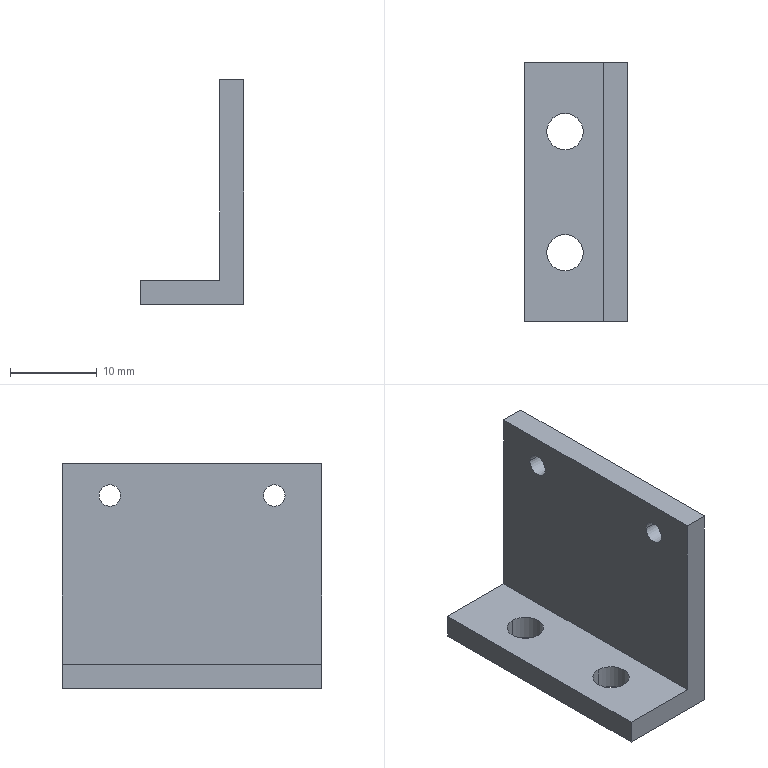Component | SolidWorks | 6G-DCSG-ZeroPointSwitchSeat-1 | 1 solid | 16 faces | box 12 x 30 x 26 mm | volume 2852 mm3 | cylinder 8 | plane 8 | commonest cylinder face diameters 2.5 x4 4.2 x4
build123d program:
from build123d import *

# Parameters (mm, degrees)
BOSS_EXTRUDE1_DEPTH = 15
SKETCH2_R           = 2.1
CUT_EXTRUDE1_DEPTH  = 30
M3_TAPPED_HOLE1_D   = 2.5
SKETCH5_W           = 7.11
SKETCH5_H           = 30
CUT_EXTRUDE2_DEPTH  = 24.497


with BuildPart() as part:
    # Sketch1 → Boss-Extrude1 (new, symmetric)
    with BuildSketch(Plane.XY):
        Polygon((-14.429, 2.972), (12.771, 2.972), (12.771, -6.228), (15.571, -6.228), (15.571, 5.772), (-14.429, 5.772), align=None)
    extrude(amount=BOSS_EXTRUDE1_DEPTH, both=True)

    # Sketch2 → Cut-Extrude1 (cut)
    with BuildSketch(Plane.ZY.offset(-12.771)):
        with Locations((-7, -1.5)):
            Circle(SKETCH2_R)
        with Locations((7, -1.5)):
            Circle(SKETCH2_R)
    extrude(amount=-CUT_EXTRUDE1_DEPTH, mode=Mode.SUBTRACT)

    # M3 Tapped Hole1 (through all)
    with Locations(Plane(origin=(-6.729, 2.972, 9.5), x_dir=(-1, 0, 0), z_dir=(0, -1, 0))):
        with Locations((0, 0), (0, 18.993)):
            Hole(M3_TAPPED_HOLE1_D / 2)

    # Sketch5 → Cut-Extrude2 (cut, through all)
    with BuildSketch(Plane.XZ.offset(-2.972)):
        with Locations((-13.984, 0)):
            Rectangle(SKETCH5_W, SKETCH5_H)
    extrude(amount=-CUT_EXTRUDE2_DEPTH, mode=Mode.SUBTRACT)


solid = part.part

# Placed as in the assembly
solid = solid.moved(Location((181.5, -79, 15.571), (90, 0, -90)))
STEP:
#1=COLOUR_RGB('',0.7922,0.8196,0.9333);
#2=FILL_AREA_STYLE_COLOUR('',#1);
#3=FILL_AREA_STYLE('',(#2));
#4=SURFACE_STYLE_FILL_AREA(#3);
#5=SURFACE_SIDE_STYLE('',(#4));
#6=SURFACE_STYLE_USAGE(.BOTH.,#5);
#7=PRESENTATION_STYLE_ASSIGNMENT((#6));
#8=CARTESIAN_POINT('',(7.373,-3.533,0.878));
#9=VERTEX_POINT('',#8);
#10=CARTESIAN_POINT('',(7.373,-3.435,0.878));
#11=VERTEX_POINT('',#10);
#12=CARTESIAN_POINT('',(7.373,-3.484,0.878));
#13=DIRECTION('',(-1.,-0.,0.));
#14=DIRECTION('',(0.,1.,0.));
#15=AXIS2_PLACEMENT_3D('',#12,#13,#14);
#16=CIRCLE('',#15,0.04921);
#17=EDGE_CURVE('',#9,#11,#16,.T.);
#18=ORIENTED_EDGE('',*,*,#17,.F.);
#19=CARTESIAN_POINT('',(7.263,-3.533,0.878));
#20=VERTEX_POINT('',#19);
#21=CARTESIAN_POINT('',(7.263,-3.533,0.878));
#22=DIRECTION('',(-1.,-0.,0.));
#23=VECTOR('',#22,39.37);
#24=LINE('',#21,#23);
#25=EDGE_CURVE('',#9,#20,#24,.T.);
#26=ORIENTED_EDGE('',*,*,#25,.T.);
#27=CARTESIAN_POINT('',(7.263,-3.435,0.878));
#28=VERTEX_POINT('',#27);
#29=CARTESIAN_POINT('',(7.263,-3.484,0.878));
#30=DIRECTION('',(-1.,-0.,0.));
#31=DIRECTION('',(0.,1.,0.));
#32=AXIS2_PLACEMENT_3D('',#29,#30,#31);
#33=CIRCLE('',#32,0.04921);
#34=EDGE_CURVE('',#20,#28,#33,.T.);
#35=ORIENTED_EDGE('',*,*,#34,.T.);
#36=CARTESIAN_POINT('',(7.263,-3.435,0.878));
#37=DIRECTION('',(-1.,-0.,0.));
#38=VECTOR('',#37,39.37);
#39=LINE('',#36,#38);
#40=EDGE_CURVE('',#11,#28,#39,.T.);
#41=ORIENTED_EDGE('',*,*,#40,.F.);
#42=EDGE_LOOP('',(#18,#26,#35,#41));
#43=FACE_OUTER_BOUND('',#42,.T.);
#44=CARTESIAN_POINT('',(7.263,-3.484,0.878));
#45=DIRECTION('',(-1.,-0.,0.));
#46=DIRECTION('',(0.,1.,0.));
#47=AXIS2_PLACEMENT_3D('',#44,#45,#46);
#48=CYLINDRICAL_SURFACE('',#47,0.04921);
#49=ADVANCED_FACE('',(#43),#48,.F.);
#50=CARTESIAN_POINT('',(7.373,-2.786,0.878));
#51=VERTEX_POINT('',#50);
#52=CARTESIAN_POINT('',(7.373,-2.687,0.878));
#53=VERTEX_POINT('',#52);
#54=CARTESIAN_POINT('',(7.373,-2.737,0.878));
#55=DIRECTION('',(-1.,-0.,0.));
#56=DIRECTION('',(0.,1.,0.));
#57=AXIS2_PLACEMENT_3D('',#54,#55,#56);
#58=CIRCLE('',#57,0.04921);
#59=EDGE_CURVE('',#51,#53,#58,.T.);
#60=ORIENTED_EDGE('',*,*,#59,.F.);
#61=CARTESIAN_POINT('',(7.263,-2.786,0.878));
#62=VERTEX_POINT('',#61);
#63=CARTESIAN_POINT('',(7.263,-2.786,0.878));
#64=DIRECTION('',(-1.,-0.,0.));
#65=VECTOR('',#64,39.37);
#66=LINE('',#63,#65);
#67=EDGE_CURVE('',#51,#62,#66,.T.);
#68=ORIENTED_EDGE('',*,*,#67,.T.);
#69=CARTESIAN_POINT('',(7.263,-2.687,0.878));
#70=VERTEX_POINT('',#69);
#71=CARTESIAN_POINT('',(7.263,-2.737,0.878));
#72=DIRECTION('',(-1.,-0.,0.));
#73=DIRECTION('',(0.,1.,0.));
#74=AXIS2_PLACEMENT_3D('',#71,#72,#73);
#75=CIRCLE('',#74,0.04921);
#76=EDGE_CURVE('',#62,#70,#75,.T.);
#77=ORIENTED_EDGE('',*,*,#76,.T.);
#78=CARTESIAN_POINT('',(7.263,-2.687,0.878));
#79=DIRECTION('',(-1.,-0.,0.));
#80=VECTOR('',#79,39.37);
#81=LINE('',#78,#80);
#82=EDGE_CURVE('',#53,#70,#81,.T.);
#83=ORIENTED_EDGE('',*,*,#82,.F.);
#84=EDGE_LOOP('',(#60,#68,#77,#83));
#85=FACE_OUTER_BOUND('',#84,.T.);
#86=CARTESIAN_POINT('',(7.263,-2.737,0.878));
#87=DIRECTION('',(-1.,-0.,0.));
#88=DIRECTION('',(0.,1.,0.));
#89=AXIS2_PLACEMENT_3D('',#86,#87,#88);
#90=CYLINDRICAL_SURFACE('',#89,0.04921);
#91=ADVANCED_FACE('',(#85),#90,.F.);
#92=CARTESIAN_POINT('',(7.087,-3.303,0.));
#93=VERTEX_POINT('',#92);
#94=CARTESIAN_POINT('',(7.087,-3.469,0.));
#95=VERTEX_POINT('',#94);
#96=CARTESIAN_POINT('',(7.087,-3.386,0.));
#97=DIRECTION('',(0.,0.,1.));
#98=DIRECTION('',(0.,-1.,0.));
#99=AXIS2_PLACEMENT_3D('',#96,#97,#98);
#100=CIRCLE('',#99,0.08268);
#101=EDGE_CURVE('',#93,#95,#100,.T.);
#102=ORIENTED_EDGE('',*,*,#101,.F.);
#103=CARTESIAN_POINT('',(7.087,-3.303,0.1102));
#104=VERTEX_POINT('',#103);
#105=CARTESIAN_POINT('',(7.087,-3.303,-1.071));
#106=DIRECTION('',(0.,0.,1.));
#107=VECTOR('',#106,39.37);
#108=LINE('',#105,#107);
#109=EDGE_CURVE('',#93,#104,#108,.T.);
#110=ORIENTED_EDGE('',*,*,#109,.T.);
#111=CARTESIAN_POINT('',(7.087,-3.469,0.1102));
#112=VERTEX_POINT('',#111);
#113=CARTESIAN_POINT('',(7.087,-3.386,0.1102));
#114=DIRECTION('',(0.,0.,1.));
#115=DIRECTION('',(0.,-1.,0.));
#116=AXIS2_PLACEMENT_3D('',#113,#114,#115);
#117=CIRCLE('',#116,0.08268);
#118=EDGE_CURVE('',#104,#112,#117,.T.);
#119=ORIENTED_EDGE('',*,*,#118,.T.);
#120=CARTESIAN_POINT('',(7.087,-3.469,-1.071));
#121=DIRECTION('',(0.,0.,1.));
#122=VECTOR('',#121,39.37);
#123=LINE('',#120,#122);
#124=EDGE_CURVE('',#95,#112,#123,.T.);
#125=ORIENTED_EDGE('',*,*,#124,.F.);
#126=EDGE_LOOP('',(#102,#110,#119,#125));
#127=FACE_OUTER_BOUND('',#126,.T.);
#128=CARTESIAN_POINT('',(7.087,-3.386,-1.071));
#129=DIRECTION('',(0.,0.,1.));
#130=DIRECTION('',(0.,-1.,0.));
#131=AXIS2_PLACEMENT_3D('',#128,#129,#130);
#132=CYLINDRICAL_SURFACE('',#131,0.08268);
#133=ADVANCED_FACE('',(#127),#132,.F.);
#134=CARTESIAN_POINT('',(7.087,-2.752,0.));
#135=VERTEX_POINT('',#134);
#136=CARTESIAN_POINT('',(7.087,-2.917,0.));
#137=VERTEX_POINT('',#136);
#138=CARTESIAN_POINT('',(7.087,-2.835,0.));
#139=DIRECTION('',(0.,0.,1.));
#140=DIRECTION('',(0.,-1.,0.));
#141=AXIS2_PLACEMENT_3D('',#138,#139,#140);
#142=CIRCLE('',#141,0.08268);
#143=EDGE_CURVE('',#135,#137,#142,.T.);
#144=ORIENTED_EDGE('',*,*,#143,.F.);
#145=CARTESIAN_POINT('',(7.087,-2.752,0.1102));
#146=VERTEX_POINT('',#145);
#147=CARTESIAN_POINT('',(7.087,-2.752,-1.071));
#148=DIRECTION('',(0.,0.,1.));
#149=VECTOR('',#148,39.37);
#150=LINE('',#147,#149);
#151=EDGE_CURVE('',#135,#146,#150,.T.);
#152=ORIENTED_EDGE('',*,*,#151,.T.);
#153=CARTESIAN_POINT('',(7.087,-2.917,0.1102));
#154=VERTEX_POINT('',#153);
#155=CARTESIAN_POINT('',(7.087,-2.835,0.1102));
#156=DIRECTION('',(0.,0.,1.));
#157=DIRECTION('',(0.,-1.,0.));
#158=AXIS2_PLACEMENT_3D('',#155,#156,#157);
#159=CIRCLE('',#158,0.08268);
#160=EDGE_CURVE('',#146,#154,#159,.T.);
#161=ORIENTED_EDGE('',*,*,#160,.T.);
#162=CARTESIAN_POINT('',(7.087,-2.917,-1.071));
#163=DIRECTION('',(0.,0.,1.));
#164=VECTOR('',#163,39.37);
#165=LINE('',#162,#164);
#166=EDGE_CURVE('',#137,#154,#165,.T.);
#167=ORIENTED_EDGE('',*,*,#166,.F.);
#168=EDGE_LOOP('',(#144,#152,#161,#167));
#169=FACE_OUTER_BOUND('',#168,.T.);
#170=CARTESIAN_POINT('',(7.087,-2.835,-1.071));
#171=DIRECTION('',(0.,0.,1.));
#172=DIRECTION('',(0.,-1.,0.));
#173=AXIS2_PLACEMENT_3D('',#170,#171,#172);
#174=CYLINDRICAL_SURFACE('',#173,0.08268);
#175=ADVANCED_FACE('',(#169),#174,.F.);
#176=CARTESIAN_POINT('',(7.087,-3.386,0.));
#177=DIRECTION('',(0.,0.,1.));
#178=DIRECTION('',(0.,-1.,0.));
#179=AXIS2_PLACEMENT_3D('',#176,#177,#178);
#180=CIRCLE('',#179,0.08268);
#181=EDGE_CURVE('',#95,#93,#180,.T.);
#182=ORIENTED_EDGE('',*,*,#181,.T.);
#183=ORIENTED_EDGE('',*,*,#101,.T.);
#184=EDGE_LOOP('',(#182,#183));
#185=FACE_BOUND('',#184,.T.);
#186=CARTESIAN_POINT('',(7.087,-2.835,0.));
#187=DIRECTION('',(0.,0.,1.));
#188=DIRECTION('',(0.,-1.,0.));
#189=AXIS2_PLACEMENT_3D('',#186,#187,#188);
#190=CIRCLE('',#189,0.08268);
#191=EDGE_CURVE('',#137,#135,#190,.T.);
#192=ORIENTED_EDGE('',*,*,#191,.T.);
#193=ORIENTED_EDGE('',*,*,#143,.T.);
#194=EDGE_LOOP('',(#192,#193));
#195=FACE_BOUND('',#194,.T.);
#196=CARTESIAN_POINT('',(6.9,-2.52,0.));
#197=VERTEX_POINT('',#196);
#198=CARTESIAN_POINT('',(7.373,-2.52,0.));
#199=VERTEX_POINT('',#198);
#200=CARTESIAN_POINT('',(6.9,-2.52,0.));
#201=DIRECTION('',(1.,0.,-0.));
#202=VECTOR('',#201,39.37);
#203=LINE('',#200,#202);
#204=EDGE_CURVE('',#197,#199,#203,.T.);
#205=ORIENTED_EDGE('',*,*,#204,.T.);
#206=CARTESIAN_POINT('',(7.373,-3.701,0.));
#207=VERTEX_POINT('',#206);
#208=CARTESIAN_POINT('',(7.373,-3.701,0.));
#209=DIRECTION('',(-0.,1.,0.));
#210=VECTOR('',#209,39.37);
#211=LINE('',#208,#210);
#212=EDGE_CURVE('',#207,#199,#211,.T.);
#213=ORIENTED_EDGE('',*,*,#212,.F.);
#214=CARTESIAN_POINT('',(6.9,-3.701,0.));
#215=VERTEX_POINT('',#214);
#216=CARTESIAN_POINT('',(6.9,-3.701,0.));
#217=DIRECTION('',(1.,0.,-0.));
#218=VECTOR('',#217,39.37);
#219=LINE('',#216,#218);
#220=EDGE_CURVE('',#215,#207,#219,.T.);
#221=ORIENTED_EDGE('',*,*,#220,.F.);
#222=CARTESIAN_POINT('',(6.9,-3.701,0.));
#223=DIRECTION('',(-0.,1.,0.));
#224=VECTOR('',#223,39.37);
#225=LINE('',#222,#224);
#226=EDGE_CURVE('',#215,#197,#225,.T.);
#227=ORIENTED_EDGE('',*,*,#226,.T.);
#228=EDGE_LOOP('',(#205,#213,#221,#227));
#229=FACE_OUTER_BOUND('',#228,.T.);
#230=CARTESIAN_POINT('',(6.9,-3.701,0.));
#231=DIRECTION('',(0.,0.,1.));
#232=DIRECTION('',(0.,-1.,0.));
#233=AXIS2_PLACEMENT_3D('',#230,#231,#232);
#234=PLANE('',#233);
#235=ADVANCED_FACE('',(#185,#195,#229),#234,.F.);
#236=CARTESIAN_POINT('',(7.373,-3.484,0.878));
#237=DIRECTION('',(-1.,-0.,0.));
#238=DIRECTION('',(0.,1.,0.));
#239=AXIS2_PLACEMENT_3D('',#236,#237,#238);
#240=CIRCLE('',#239,0.04921);
#241=EDGE_CURVE('',#11,#9,#240,.T.);
#242=ORIENTED_EDGE('',*,*,#241,.T.);
#243=ORIENTED_EDGE('',*,*,#17,.T.);
#244=EDGE_LOOP('',(#242,#243));
#245=FACE_BOUND('',#244,.T.);
#246=CARTESIAN_POINT('',(7.373,-2.737,0.878));
#247=DIRECTION('',(-1.,-0.,0.));
#248=DIRECTION('',(0.,1.,0.));
#249=AXIS2_PLACEMENT_3D('',#246,#247,#248);
#250=CIRCLE('',#249,0.04921);
#251=EDGE_CURVE('',#53,#51,#250,.T.);
#252=ORIENTED_EDGE('',*,*,#251,.T.);
#253=ORIENTED_EDGE('',*,*,#59,.T.);
#254=EDGE_LOOP('',(#252,#253));
#255=FACE_BOUND('',#254,.T.);
#256=CARTESIAN_POINT('',(7.373,-2.52,1.024));
#257=VERTEX_POINT('',#256);
#258=CARTESIAN_POINT('',(7.373,-2.52,1.181));
#259=DIRECTION('',(0.,0.,1.));
#260=VECTOR('',#259,39.37);
#261=LINE('',#258,#260);
#262=EDGE_CURVE('',#199,#257,#261,.T.);
#263=ORIENTED_EDGE('',*,*,#262,.T.);
#264=CARTESIAN_POINT('',(7.373,-3.701,1.024));
#265=VERTEX_POINT('',#264);
#266=CARTESIAN_POINT('',(7.373,-3.701,1.024));
#267=DIRECTION('',(0.,-1.,0.));
#268=VECTOR('',#267,39.37);
#269=LINE('',#266,#268);
#270=EDGE_CURVE('',#257,#265,#269,.T.);
#271=ORIENTED_EDGE('',*,*,#270,.T.);
#272=CARTESIAN_POINT('',(7.373,-3.701,1.181));
#273=DIRECTION('',(0.,0.,1.));
#274=VECTOR('',#273,39.37);
#275=LINE('',#272,#274);
#276=EDGE_CURVE('',#207,#265,#275,.T.);
#277=ORIENTED_EDGE('',*,*,#276,.F.);
#278=ORIENTED_EDGE('',*,*,#212,.T.);
#279=EDGE_LOOP('',(#263,#271,#277,#278));
#280=FACE_OUTER_BOUND('',#279,.T.);
#281=CARTESIAN_POINT('',(7.373,-3.701,1.181));
#282=DIRECTION('',(-1.,-0.,0.));
#283=DIRECTION('',(-0.,1.,0.));
#284=AXIS2_PLACEMENT_3D('',#281,#282,#283);
#285=PLANE('',#284);
#286=ADVANCED_FACE('',(#245,#255,#280),#285,.F.);
#287=CARTESIAN_POINT('',(7.263,-3.484,0.878));
#288=DIRECTION('',(-1.,-0.,0.));
#289=DIRECTION('',(0.,1.,0.));
#290=AXIS2_PLACEMENT_3D('',#287,#288,#289);
#291=CIRCLE('',#290,0.04921);
#292=EDGE_CURVE('',#28,#20,#291,.T.);
#293=ORIENTED_EDGE('',*,*,#292,.F.);
#294=ORIENTED_EDGE('',*,*,#34,.F.);
#295=EDGE_LOOP('',(#293,#294));
#296=FACE_BOUND('',#295,.T.);
#297=CARTESIAN_POINT('',(7.263,-2.737,0.878));
#298=DIRECTION('',(-1.,-0.,0.));
#299=DIRECTION('',(0.,1.,0.));
#300=AXIS2_PLACEMENT_3D('',#297,#298,#299);
#301=CIRCLE('',#300,0.04921);
#302=EDGE_CURVE('',#70,#62,#301,.T.);
#303=ORIENTED_EDGE('',*,*,#302,.F.);
#304=ORIENTED_EDGE('',*,*,#76,.F.);
#305=EDGE_LOOP('',(#303,#304));
#306=FACE_BOUND('',#305,.T.);
#307=CARTESIAN_POINT('',(7.263,-3.701,1.024));
#308=VERTEX_POINT('',#307);
#309=CARTESIAN_POINT('',(7.263,-3.701,0.1102));
#310=VERTEX_POINT('',#309);
#311=CARTESIAN_POINT('',(7.263,-3.701,1.181));
#312=DIRECTION('',(-0.,-0.,-1.));
#313=VECTOR('',#312,39.37);
#314=LINE('',#311,#313);
#315=EDGE_CURVE('',#308,#310,#314,.T.);
#316=ORIENTED_EDGE('',*,*,#315,.F.);
#317=CARTESIAN_POINT('',(7.263,-2.52,1.024));
#318=VERTEX_POINT('',#317);
#319=CARTESIAN_POINT('',(7.263,-3.701,1.024));
#320=DIRECTION('',(0.,-1.,0.));
#321=VECTOR('',#320,39.37);
#322=LINE('',#319,#321);
#323=EDGE_CURVE('',#318,#308,#322,.T.);
#324=ORIENTED_EDGE('',*,*,#323,.F.);
#325=CARTESIAN_POINT('',(7.263,-2.52,0.1102));
#326=VERTEX_POINT('',#325);
#327=CARTESIAN_POINT('',(7.263,-2.52,1.181));
#328=DIRECTION('',(-0.,-0.,-1.));
#329=VECTOR('',#328,39.37);
#330=LINE('',#327,#329);
#331=EDGE_CURVE('',#318,#326,#330,.T.);
#332=ORIENTED_EDGE('',*,*,#331,.T.);
#333=CARTESIAN_POINT('',(7.263,-3.701,0.1102));
#334=DIRECTION('',(-0.,1.,0.));
#335=VECTOR('',#334,39.37);
#336=LINE('',#333,#335);
#337=EDGE_CURVE('',#310,#326,#336,.T.);
#338=ORIENTED_EDGE('',*,*,#337,.F.);
#339=EDGE_LOOP('',(#316,#324,#332,#338));
#340=FACE_OUTER_BOUND('',#339,.T.);
#341=CARTESIAN_POINT('',(7.263,-3.701,1.181));
#342=DIRECTION('',(1.,0.,-0.));
#343=DIRECTION('',(0.,0.,1.));
#344=AXIS2_PLACEMENT_3D('',#341,#342,#343);
#345=PLANE('',#344);
#346=ADVANCED_FACE('',(#296,#306,#340),#345,.F.);
#347=CARTESIAN_POINT('',(7.087,-3.386,0.1102));
#348=DIRECTION('',(0.,0.,1.));
#349=DIRECTION('',(0.,-1.,0.));
#350=AXIS2_PLACEMENT_3D('',#347,#348,#349);
#351=CIRCLE('',#350,0.08268);
#352=EDGE_CURVE('',#112,#104,#351,.T.);
#353=ORIENTED_EDGE('',*,*,#352,.F.);
#354=ORIENTED_EDGE('',*,*,#118,.F.);
#355=EDGE_LOOP('',(#353,#354));
#356=FACE_BOUND('',#355,.T.);
#357=CARTESIAN_POINT('',(7.087,-2.835,0.1102));
#358=DIRECTION('',(0.,0.,1.));
#359=DIRECTION('',(0.,-1.,0.));
#360=AXIS2_PLACEMENT_3D('',#357,#358,#359);
#361=CIRCLE('',#360,0.08268);
#362=EDGE_CURVE('',#154,#146,#361,.T.);
#363=ORIENTED_EDGE('',*,*,#362,.F.);
#364=ORIENTED_EDGE('',*,*,#160,.F.);
#365=EDGE_LOOP('',(#363,#364));
#366=FACE_BOUND('',#365,.T.);
#367=CARTESIAN_POINT('',(6.9,-2.52,0.1102));
#368=VERTEX_POINT('',#367);
#369=CARTESIAN_POINT('',(6.9,-2.52,0.1102));
#370=DIRECTION('',(-1.,-0.,0.));
#371=VECTOR('',#370,39.37);
#372=LINE('',#369,#371);
#373=EDGE_CURVE('',#326,#368,#372,.T.);
#374=ORIENTED_EDGE('',*,*,#373,.T.);
#375=CARTESIAN_POINT('',(6.9,-3.701,0.1102));
#376=VERTEX_POINT('',#375);
#377=CARTESIAN_POINT('',(6.9,-3.701,0.1102));
#378=DIRECTION('',(-0.,1.,0.));
#379=VECTOR('',#378,39.37);
#380=LINE('',#377,#379);
#381=EDGE_CURVE('',#376,#368,#380,.T.);
#382=ORIENTED_EDGE('',*,*,#381,.F.);
#383=CARTESIAN_POINT('',(6.9,-3.701,0.1102));
#384=DIRECTION('',(-1.,-0.,0.));
#385=VECTOR('',#384,39.37);
#386=LINE('',#383,#385);
#387=EDGE_CURVE('',#310,#376,#386,.T.);
#388=ORIENTED_EDGE('',*,*,#387,.F.);
#389=ORIENTED_EDGE('',*,*,#337,.T.);
#390=EDGE_LOOP('',(#374,#382,#388,#389));
#391=FACE_OUTER_BOUND('',#390,.T.);
#392=CARTESIAN_POINT('',(6.9,-3.701,0.1102));
#393=DIRECTION('',(-0.,-0.,-1.));
#394=DIRECTION('',(1.,0.,-0.));
#395=AXIS2_PLACEMENT_3D('',#392,#393,#394);
#396=PLANE('',#395);
#397=ADVANCED_FACE('',(#356,#366,#391),#396,.F.);
#398=CARTESIAN_POINT('',(6.9,-2.52,0.1102));
#399=DIRECTION('',(0.,0.,-1.));
#400=VECTOR('',#399,39.37);
#401=LINE('',#398,#400);
#402=EDGE_CURVE('',#368,#197,#401,.T.);
#403=ORIENTED_EDGE('',*,*,#402,.T.);
#404=ORIENTED_EDGE('',*,*,#226,.F.);
#405=CARTESIAN_POINT('',(6.9,-3.701,0.1102));
#406=DIRECTION('',(0.,0.,-1.));
#407=VECTOR('',#406,39.37);
#408=LINE('',#405,#407);
#409=EDGE_CURVE('',#376,#215,#408,.T.);
#410=ORIENTED_EDGE('',*,*,#409,.F.);
#411=ORIENTED_EDGE('',*,*,#381,.T.);
#412=EDGE_LOOP('',(#403,#404,#410,#411));
#413=FACE_OUTER_BOUND('',#412,.T.);
#414=CARTESIAN_POINT('',(6.9,-3.701,0.1102));
#415=DIRECTION('',(1.,0.,-0.));
#416=DIRECTION('',(0.,-1.,0.));
#417=AXIS2_PLACEMENT_3D('',#414,#415,#416);
#418=PLANE('',#417);
#419=ADVANCED_FACE('',(#413),#418,.F.);
#420=ORIENTED_EDGE('',*,*,#276,.T.);
#421=CARTESIAN_POINT('',(7.373,-3.701,1.024));
#422=DIRECTION('',(-1.,-0.,0.));
#423=VECTOR('',#422,39.37);
#424=LINE('',#421,#423);
#425=EDGE_CURVE('',#265,#308,#424,.T.);
#426=ORIENTED_EDGE('',*,*,#425,.T.);
#427=ORIENTED_EDGE('',*,*,#315,.T.);
#428=ORIENTED_EDGE('',*,*,#387,.T.);
#429=ORIENTED_EDGE('',*,*,#409,.T.);
#430=ORIENTED_EDGE('',*,*,#220,.T.);
#431=EDGE_LOOP('',(#420,#426,#427,#428,#429,#430));
#432=FACE_OUTER_BOUND('',#431,.T.);
#433=CARTESIAN_POINT('',(7.146,-3.701,0.613));
#434=DIRECTION('',(-0.,1.,0.));
#435=DIRECTION('',(0.,0.,1.));
#436=AXIS2_PLACEMENT_3D('',#433,#434,#435);
#437=PLANE('',#436);
#438=ADVANCED_FACE('',(#432),#437,.F.);
#439=CARTESIAN_POINT('',(7.373,-2.52,1.024));
#440=DIRECTION('',(-1.,-0.,0.));
#441=VECTOR('',#440,39.37);
#442=LINE('',#439,#441);
#443=EDGE_CURVE('',#257,#318,#442,.T.);
#444=ORIENTED_EDGE('',*,*,#443,.F.);
#445=ORIENTED_EDGE('',*,*,#262,.F.);
#446=ORIENTED_EDGE('',*,*,#204,.F.);
#447=ORIENTED_EDGE('',*,*,#402,.F.);
#448=ORIENTED_EDGE('',*,*,#373,.F.);
#449=ORIENTED_EDGE('',*,*,#331,.F.);
#450=EDGE_LOOP('',(#444,#445,#446,#447,#448,#449));
#451=FACE_OUTER_BOUND('',#450,.T.);
#452=CARTESIAN_POINT('',(7.146,-2.52,0.613));
#453=DIRECTION('',(-0.,1.,0.));
#454=DIRECTION('',(0.,0.,1.));
#455=AXIS2_PLACEMENT_3D('',#452,#453,#454);
#456=PLANE('',#455);
#457=ADVANCED_FACE('',(#451),#456,.T.);
#458=ORIENTED_EDGE('',*,*,#151,.F.);
#459=ORIENTED_EDGE('',*,*,#191,.F.);
#460=ORIENTED_EDGE('',*,*,#166,.T.);
#461=ORIENTED_EDGE('',*,*,#362,.T.);
#462=EDGE_LOOP('',(#458,#459,#460,#461));
#463=FACE_OUTER_BOUND('',#462,.T.);
#464=CARTESIAN_POINT('',(7.087,-2.835,-1.071));
#465=DIRECTION('',(0.,0.,1.));
#466=DIRECTION('',(0.,-1.,0.));
#467=AXIS2_PLACEMENT_3D('',#464,#465,#466);
#468=CYLINDRICAL_SURFACE('',#467,0.08268);
#469=ADVANCED_FACE('',(#463),#468,.F.);
#470=ORIENTED_EDGE('',*,*,#109,.F.);
#471=ORIENTED_EDGE('',*,*,#181,.F.);
#472=ORIENTED_EDGE('',*,*,#124,.T.);
#473=ORIENTED_EDGE('',*,*,#352,.T.);
#474=EDGE_LOOP('',(#470,#471,#472,#473));
#475=FACE_OUTER_BOUND('',#474,.T.);
#476=CARTESIAN_POINT('',(7.087,-3.386,-1.071));
#477=DIRECTION('',(0.,0.,1.));
#478=DIRECTION('',(0.,-1.,0.));
#479=AXIS2_PLACEMENT_3D('',#476,#477,#478);
#480=CYLINDRICAL_SURFACE('',#479,0.08268);
#481=ADVANCED_FACE('',(#475),#480,.F.);
#482=ORIENTED_EDGE('',*,*,#67,.F.);
#483=ORIENTED_EDGE('',*,*,#251,.F.);
#484=ORIENTED_EDGE('',*,*,#82,.T.);
#485=ORIENTED_EDGE('',*,*,#302,.T.);
#486=EDGE_LOOP('',(#482,#483,#484,#485));
#487=FACE_OUTER_BOUND('',#486,.T.);
#488=CARTESIAN_POINT('',(7.263,-2.737,0.878));
#489=DIRECTION('',(-1.,-0.,0.));
#490=DIRECTION('',(0.,1.,0.));
#491=AXIS2_PLACEMENT_3D('',#488,#489,#490);
#492=CYLINDRICAL_SURFACE('',#491,0.04921);
#493=ADVANCED_FACE('',(#487),#492,.F.);
#494=ORIENTED_EDGE('',*,*,#25,.F.);
#495=ORIENTED_EDGE('',*,*,#241,.F.);
#496=ORIENTED_EDGE('',*,*,#40,.T.);
#497=ORIENTED_EDGE('',*,*,#292,.T.);
#498=EDGE_LOOP('',(#494,#495,#496,#497));
#499=FACE_OUTER_BOUND('',#498,.T.);
#500=CARTESIAN_POINT('',(7.263,-3.484,0.878));
#501=DIRECTION('',(-1.,-0.,0.));
#502=DIRECTION('',(0.,1.,0.));
#503=AXIS2_PLACEMENT_3D('',#500,#501,#502);
#504=CYLINDRICAL_SURFACE('',#503,0.04921);
#505=ADVANCED_FACE('',(#499),#504,.F.);
#506=ORIENTED_EDGE('',*,*,#323,.T.);
#507=ORIENTED_EDGE('',*,*,#425,.F.);
#508=ORIENTED_EDGE('',*,*,#270,.F.);
#509=ORIENTED_EDGE('',*,*,#443,.T.);
#510=EDGE_LOOP('',(#506,#507,#508,#509));
#511=FACE_OUTER_BOUND('',#510,.T.);
#512=CARTESIAN_POINT('',(7.373,-3.701,1.024));
#513=DIRECTION('',(0.,0.,-1.));
#514=DIRECTION('',(-0.,1.,0.));
#515=AXIS2_PLACEMENT_3D('',#512,#513,#514);
#516=PLANE('',#515);
#517=ADVANCED_FACE('',(#511),#516,.F.);
#518=CLOSED_SHELL('',(#49,#91,#133,#175,#235,#286,#346,#397,#419,#438,#457,#469,#481,#493,#505,#517));
#519=MANIFOLD_SOLID_BREP('',#518);
#520=STYLED_ITEM('',(#7),#519);
#521=PRESENTATION_LAYER_ASSIGNMENT('','',(#520));
#522=(LENGTH_UNIT()NAMED_UNIT(*)SI_UNIT($,.METRE.));
#523=LENGTH_MEASURE_WITH_UNIT(LENGTH_MEASURE(0.0254),#522);
#524=DIMENSIONAL_EXPONENTS(1.,0.,0.,0.,0.,0.,0.);
#525=(CONVERSION_BASED_UNIT('',#523)LENGTH_UNIT()NAMED_UNIT(#524));
#526=UNCERTAINTY_MEASURE_WITH_UNIT(LENGTH_MEASURE(0.00001),#525,'','');
#527=(NAMED_UNIT(*)PLANE_ANGLE_UNIT()SI_UNIT($,.RADIAN.));
#528=(NAMED_UNIT(*)SI_UNIT($,.STERADIAN.)SOLID_ANGLE_UNIT());
#529=(GEOMETRIC_REPRESENTATION_CONTEXT(3)GLOBAL_UNCERTAINTY_ASSIGNED_CONTEXT((#526))GLOBAL_UNIT_ASSIGNED_CONTEXT((#525,#527,#528))REPRESENTATION_CONTEXT('',''));
#530=MECHANICAL_DESIGN_GEOMETRIC_PRESENTATION_REPRESENTATION('',(#520),#529);
#531=CARTESIAN_POINT('',(0.,0.,0.));
#532=DIRECTION('',(0.,0.,1.));
#533=DIRECTION('',(1.,0.,0.));
#534=AXIS2_PLACEMENT_3D('',#531,#532,#533);
#535=(LENGTH_UNIT()NAMED_UNIT(*)SI_UNIT($,.METRE.));
#536=LENGTH_MEASURE_WITH_UNIT(LENGTH_MEASURE(0.0254),#535);
#537=DIMENSIONAL_EXPONENTS(1.,0.,0.,0.,0.,0.,0.);
#538=(CONVERSION_BASED_UNIT('',#536)LENGTH_UNIT()NAMED_UNIT(#537));
#539=UNCERTAINTY_MEASURE_WITH_UNIT(LENGTH_MEASURE(0.00001),#538,'','');
#540=(NAMED_UNIT(*)PLANE_ANGLE_UNIT()SI_UNIT($,.RADIAN.));
#541=(NAMED_UNIT(*)SI_UNIT($,.STERADIAN.)SOLID_ANGLE_UNIT());
#542=(GEOMETRIC_REPRESENTATION_CONTEXT(3)GLOBAL_UNCERTAINTY_ASSIGNED_CONTEXT((#539))GLOBAL_UNIT_ASSIGNED_CONTEXT((#538,#540,#541))REPRESENTATION_CONTEXT('',''));
#543=ADVANCED_BREP_SHAPE_REPRESENTATION('',(#519,#534),#542);